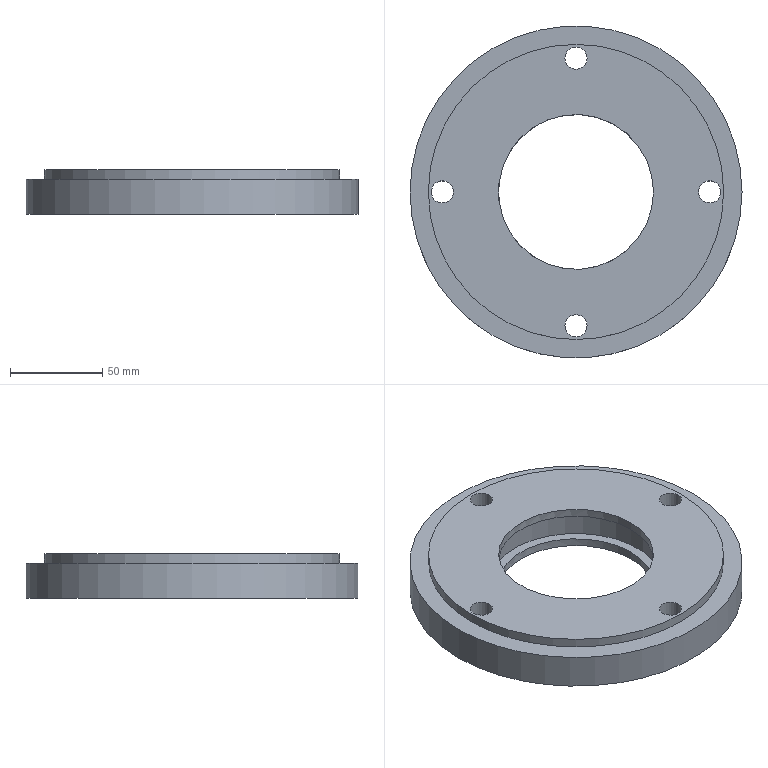Component | NX | CA6140-ZHUZHOU-DUANGAIZUO | 1 solid | 22 faces | volume 414668 mm3 | cylinder 13 | plane 9 | commonest cylinder face diameters 18 x4 12 x4 84 x2 160 x1 180 x1 94 x1